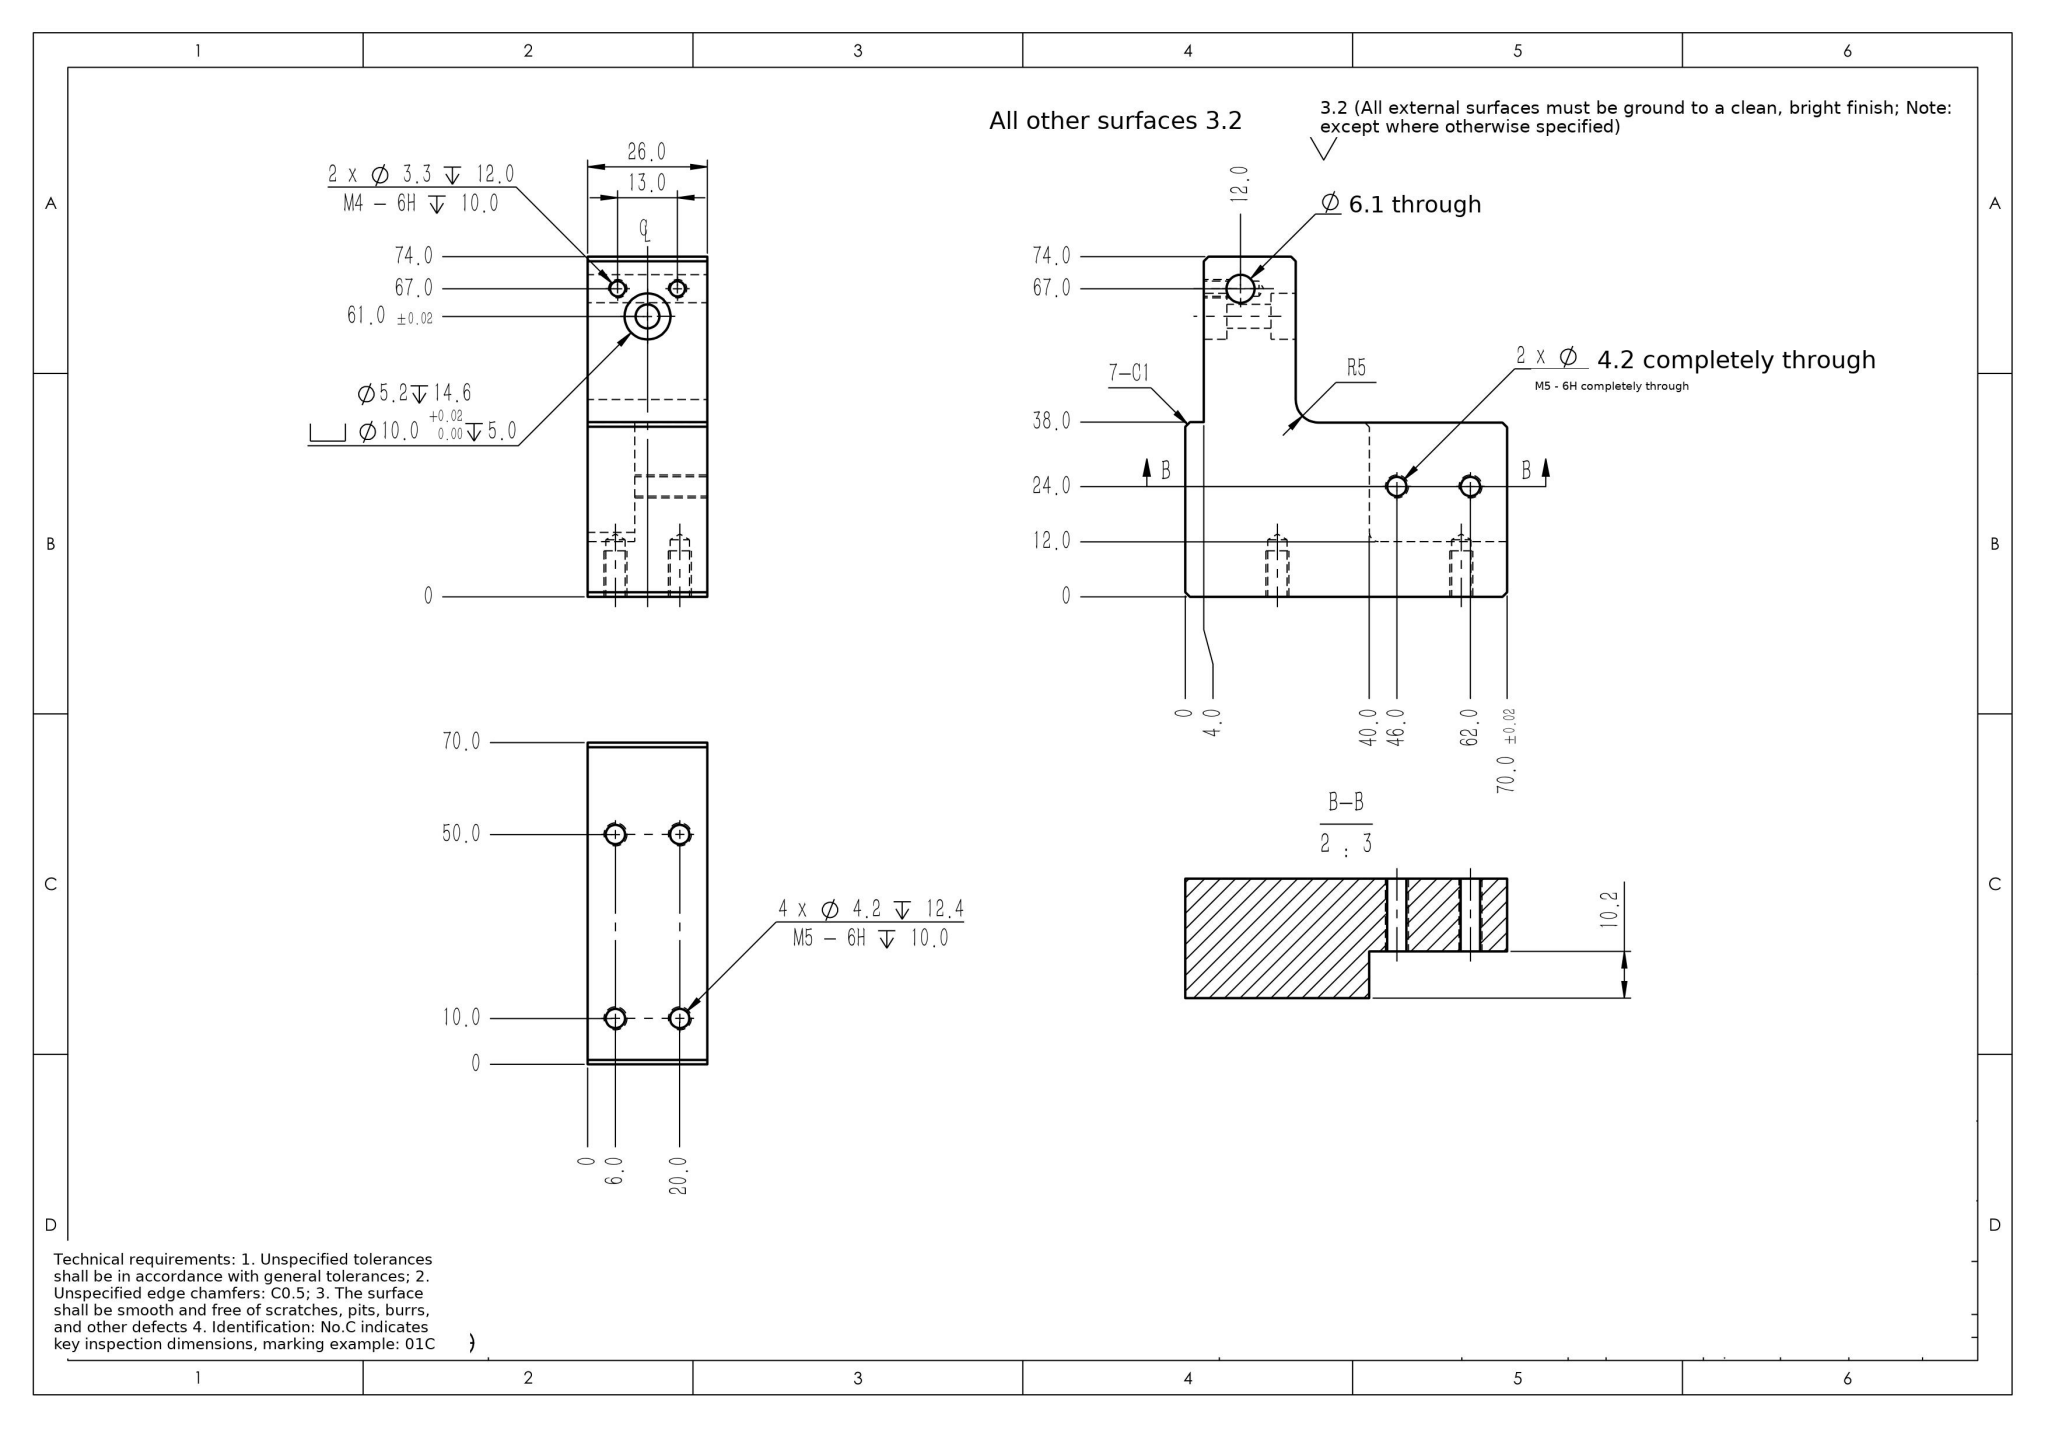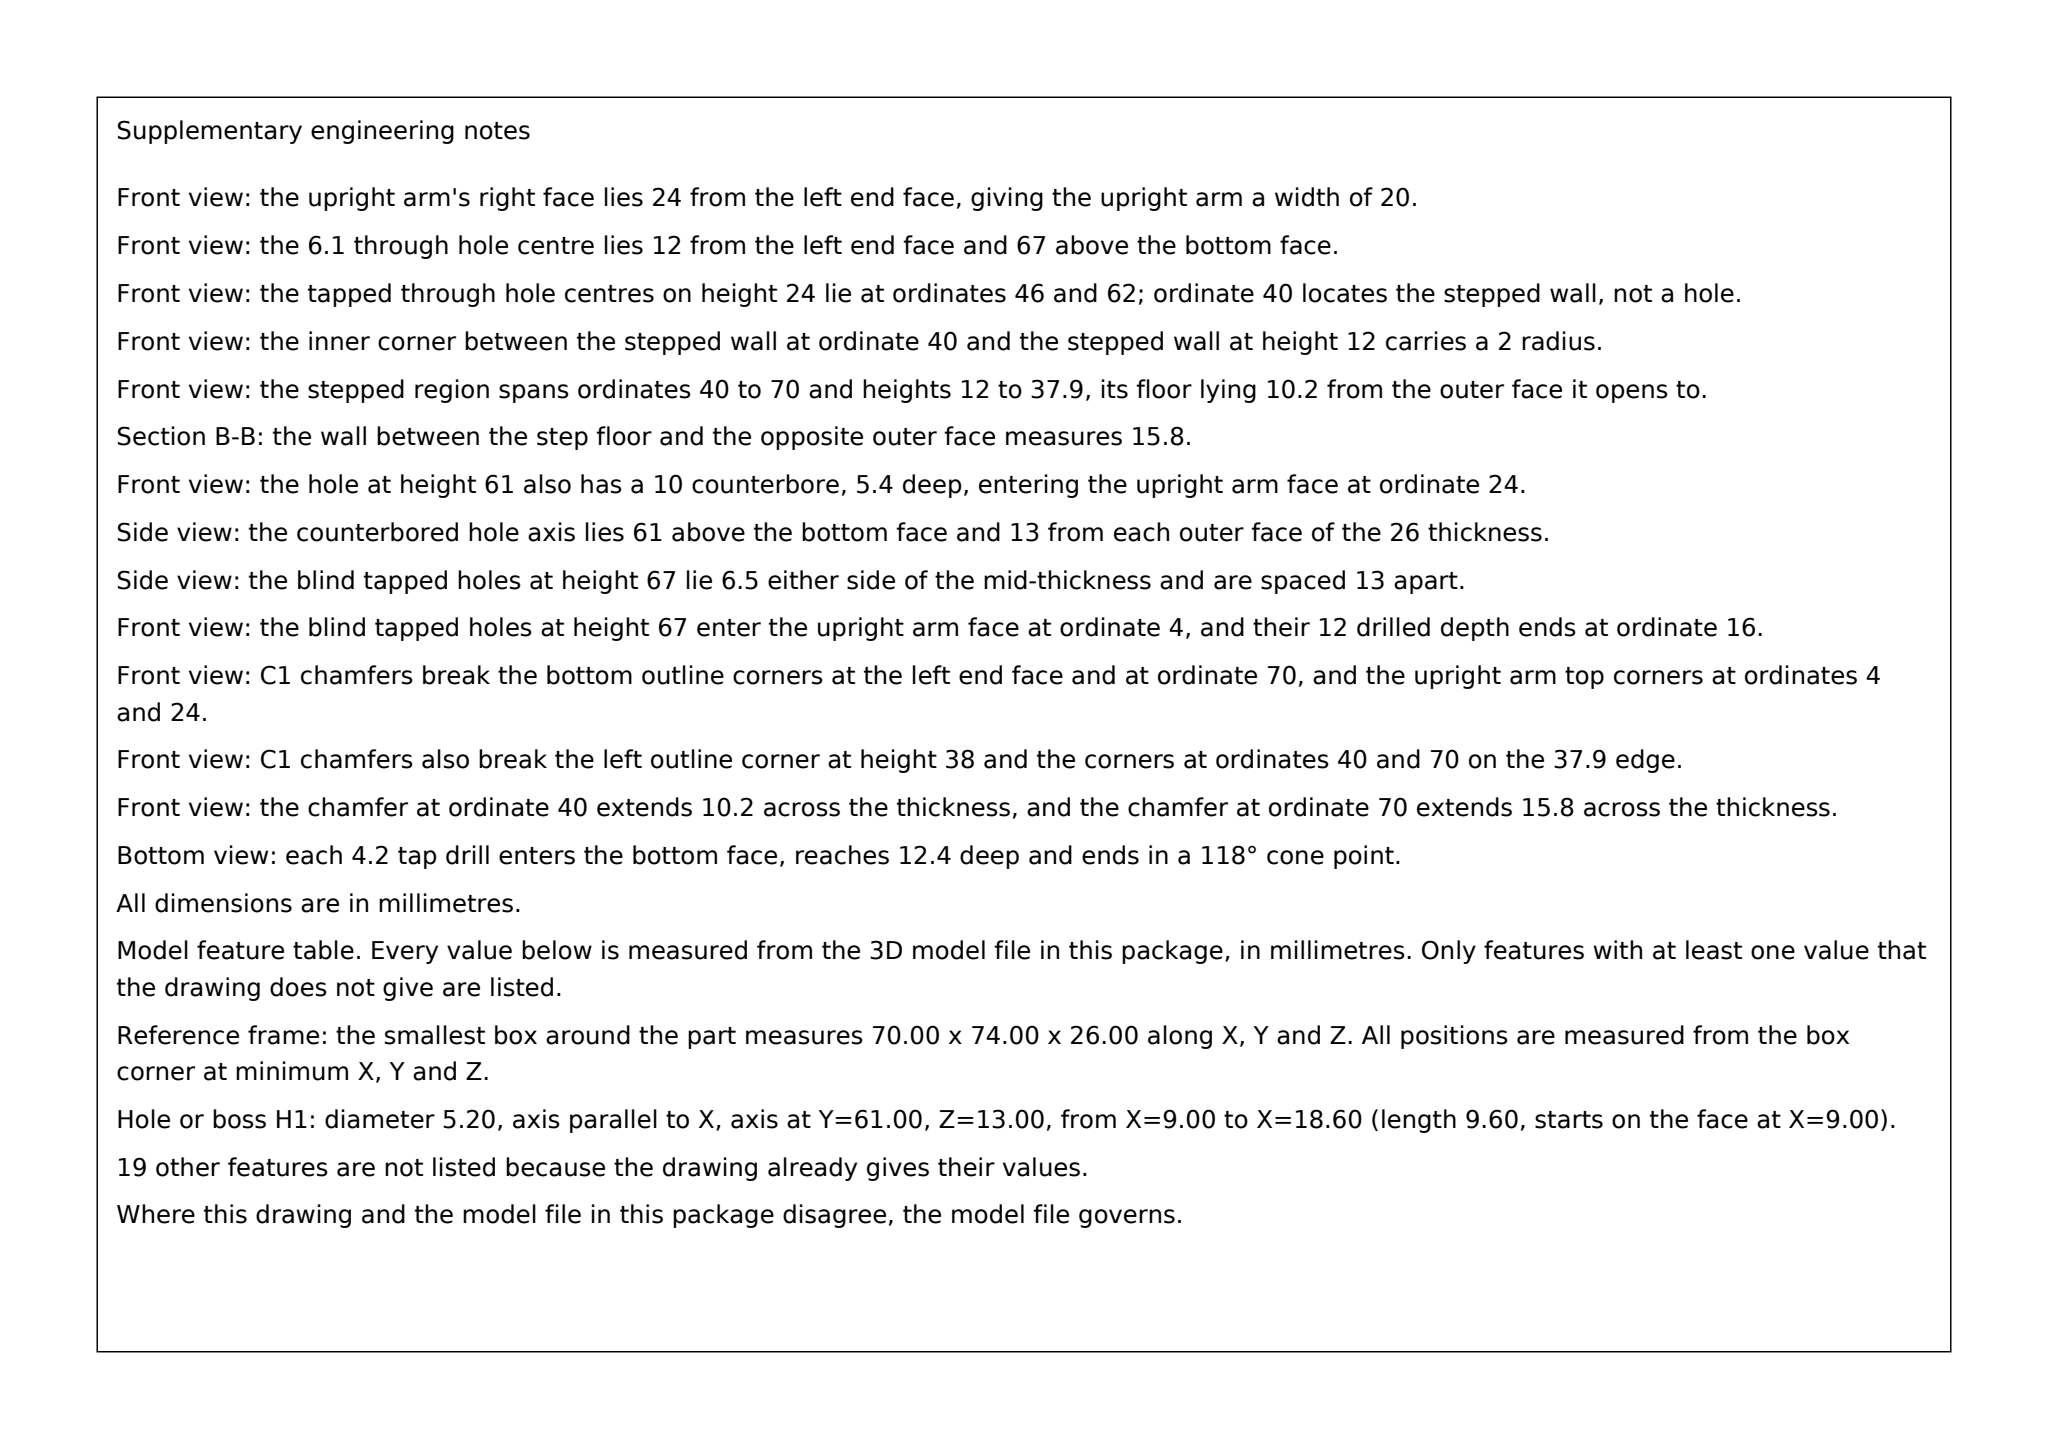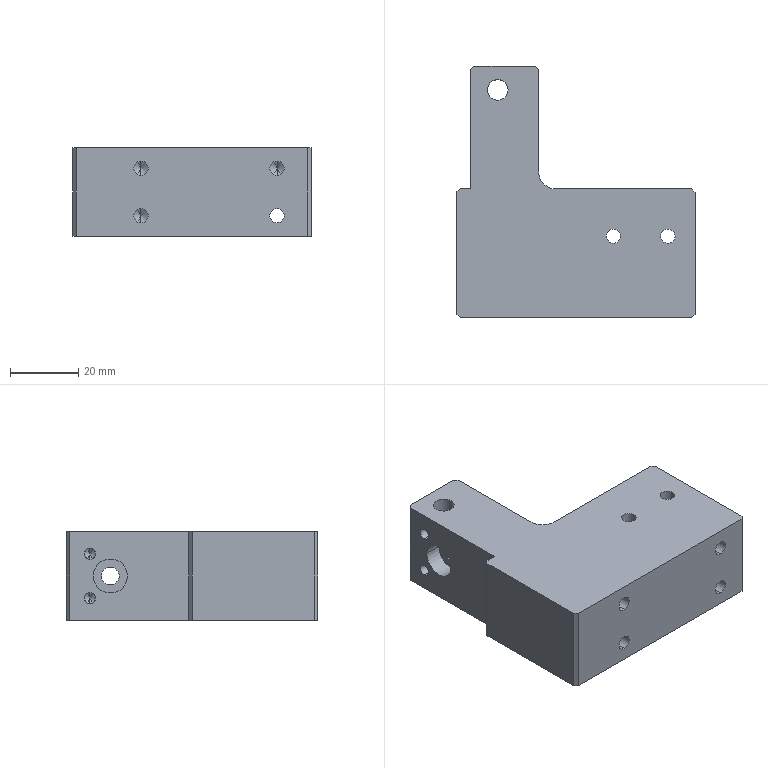Part | SolidWorks | mm | 1 solid | 62 faces | box 70 x 74 x 26 mm | volume 76877 mm3 | cylinder 30 | plane 22 | cone 10 | commonest cylinder face diameters 4.2 x12 3.3 x8 10 x5 5.2 x2 6.1 x2 4 x1
Drawing notes:
2 x M4-6H HOLES AT 6.5 FROM EA EDGE OF 26.0 FACE (13.0 APART) | from the solid: Ø3.3 x-axis holes at z=6.5 and z=19.5 on 26.0 wide face; y=67.0
ADD Ø4.0 DP 10.2 THRU STEP: X=42.0 FROM LH EDGE, Y=14.0 FROM BOTTOM | from the solid: cylinder [4.0,'z',[42.0,14.0],10.2]; step face z=10.2, bbox 70x74x26
UPRIGHT WIDTH 24.0 FROM LEFT EDGE (0) TO R5 TANGENT FACE | from the solid: axis_planes x=0.0 and x=24.0 define vertical leg faces; R5 fillet tangent at x=24.0
build123d program:
from build123d import *

# Parameters (mm, degrees)
SKETCH1_W                                       = 70
SKETCH1_H                                       = 74
BOSS_EXTRUDE1_DEPTH                             = 13
SKETCH2_W                                       = 46
SKETCH2_H                                       = 36.1
SKETCH2_W_2                                     = 4
SKETCH2_H_2                                     = 36
CUT_EXTRUDE1_DEPTH                              = 86.889
SKETCH4_R                                       = 3.05
CUT_EXTRUDE3_DEPTH                              = 86.889
SKETCH5_R                                       = 5
CUT_EXTRUDE4_DEPTH                              = 5
SKETCH6_R                                       = 2.6
CUT_EXTRUDE5_DEPTH                              = 101.005
SKETCH12_W                                      = 30
SKETCH12_H                                      = 25.9
CUT_EXTRUDE6_DEPTH                              = 10.2
M4_TAPPED_HOLE1_D                               = 3.3
M4_TAPPED_HOLE1_DEPTH                           = 12
M4_TAPPED_HOLE1_TIP                             = 0.9914
M5_TAPPED_HOLE1_D                               = 4.2
M5_TAPPED_HOLE1_DEPTH                           = 12.4
M5_TAPPED_HOLE1_TIP                             = 1.262
M5_TAPPED_HOLE2_D                               = 4.2
FILLET1_R                                       = 5
FILLET2_R                                       = 2
CHAMFER1_SIZE                                   = 1
M5_HEX_SOCKET_HEAD_CAP_SCREW_CBORE1_D           = 5.2
M5_HEX_SOCKET_HEAD_CAP_SCREW_CBORE1_CBORE_D     = 10
M5_HEX_SOCKET_HEAD_CAP_SCREW_CBORE1_CBORE_DEPTH = 5.4


with BuildPart() as part:
    # Sketch1 → Boss-Extrude1 (new, symmetric)
    with BuildSketch(Plane.XY):
        with Locations((0, 37)):
            Rectangle(SKETCH1_W, SKETCH1_H)
    extrude(amount=BOSS_EXTRUDE1_DEPTH, both=True)

    # Sketch2 → Cut-Extrude1 (cut, through all)
    with BuildSketch(Plane.XY.offset(13)):
        with Locations((12, 55.95)):
            Rectangle(SKETCH2_W, SKETCH2_H)
        with Locations((-33, 56)):
            Rectangle(SKETCH2_W_2, SKETCH2_H_2)
    extrude(amount=-CUT_EXTRUDE1_DEPTH, mode=Mode.SUBTRACT)

    # Sketch4 → Cut-Extrude3 (cut, through all)
    with BuildSketch(Plane(origin=(0, 0, -13), x_dir=(-1, 0, 0), z_dir=(0, 0, -1))):
        with Locations((23, 67)):
            Circle(SKETCH4_R)
    extrude(amount=-CUT_EXTRUDE3_DEPTH, mode=Mode.SUBTRACT)

    # Sketch5 → Cut-Extrude4 (cut)
    with BuildSketch(Plane.ZY.offset(31)):
        with Locations(Location((0, 61, 0), (0, 0, 270))):
            Circle(SKETCH5_R)
    extrude(amount=-CUT_EXTRUDE4_DEPTH, mode=Mode.SUBTRACT)

    # Sketch6 → Cut-Extrude5 (cut, through all)
    with BuildSketch(Plane.ZY.offset(31)):
        with Locations(Location((0, 61, 0), (0, 0, 270))):
            Circle(SKETCH6_R)
    extrude(amount=-CUT_EXTRUDE5_DEPTH, mode=Mode.SUBTRACT)

    # Sketch12 → Cut-Extrude6 (cut)
    with BuildSketch(Plane(origin=(0, 0, -13), x_dir=(-1, 0, 0), z_dir=(0, 0, -1))):
        with Locations((-20, 24.95)):
            Rectangle(SKETCH12_W, SKETCH12_H)
    extrude(amount=-CUT_EXTRUDE6_DEPTH, mode=Mode.SUBTRACT)

    # M4 Tapped Hole1
    with Locations(Plane.ZY.offset(31)):
        with Locations((-6.5, 67), (6.5, 67)):
            Hole(M4_TAPPED_HOLE1_D / 2, depth=M4_TAPPED_HOLE1_DEPTH)
            with Locations((0, 0, -(M4_TAPPED_HOLE1_DEPTH + M4_TAPPED_HOLE1_TIP / 2))):  # 118° drill point
                Cone(0, M4_TAPPED_HOLE1_D / 2, M4_TAPPED_HOLE1_TIP, mode=Mode.SUBTRACT)

    # M5 Tapped Hole1
    with Locations(Plane(origin=(0, 0, 0), x_dir=(-1, 0, 0), z_dir=(0, -1, 0))):
        with Locations((15, 7), (15, -7), (-25, 7), (-25, -7)):
            Hole(M5_TAPPED_HOLE1_D / 2, depth=M5_TAPPED_HOLE1_DEPTH)
            with Locations((0, 0, -(M5_TAPPED_HOLE1_DEPTH + M5_TAPPED_HOLE1_TIP / 2))):  # 118° drill point
                Cone(0, M5_TAPPED_HOLE1_D / 2, M5_TAPPED_HOLE1_TIP, mode=Mode.SUBTRACT)

    # M5 Tapped Hole2 (through all)
    with Locations(Plane(origin=(0, 0, -2.8), x_dir=(-1, 0, 0), z_dir=(0, 0, -1))):
        with Locations((-11, 24), (-27, 24)):
            Hole(M5_TAPPED_HOLE2_D / 2)

    # Fillet1
    fillet1_edges = [part.edges().sort_by_distance(p)[0] for p in [
        (-11, 37.9, 0),
    ]]
    fillet(fillet1_edges, radius=FILLET1_R)

    # Fillet2
    fillet2_edges = [part.edges().sort_by_distance(p)[0] for p in [
        (5, 12, -7.9),
    ]]
    fillet(fillet2_edges, radius=FILLET2_R)

    # Chamfer1
    chamfer1_edges = [part.edges().sort_by_distance(p)[0] for p in [
        (-11, 74, 0),
        (-35, 38, 0),
        (-31, 74, 0),
        (35, 37.9, 5.1),
        (5, 37.9, -7.9),
        (-35, 0, 0),
        (35, 0, 0),
    ]]
    chamfer(chamfer1_edges, length=CHAMFER1_SIZE)

    # M5 Hex Socket Head Cap Screw CBORE1 (through all)
    with Locations(Plane(origin=(-11, 0, 0), x_dir=(0, 0, -1), z_dir=(1, 0, 0))):
        with Locations((0, 61)):
            CounterBoreHole(M5_HEX_SOCKET_HEAD_CAP_SCREW_CBORE1_D / 2, M5_HEX_SOCKET_HEAD_CAP_SCREW_CBORE1_CBORE_D / 2, M5_HEX_SOCKET_HEAD_CAP_SCREW_CBORE1_CBORE_DEPTH)


solid = part.part